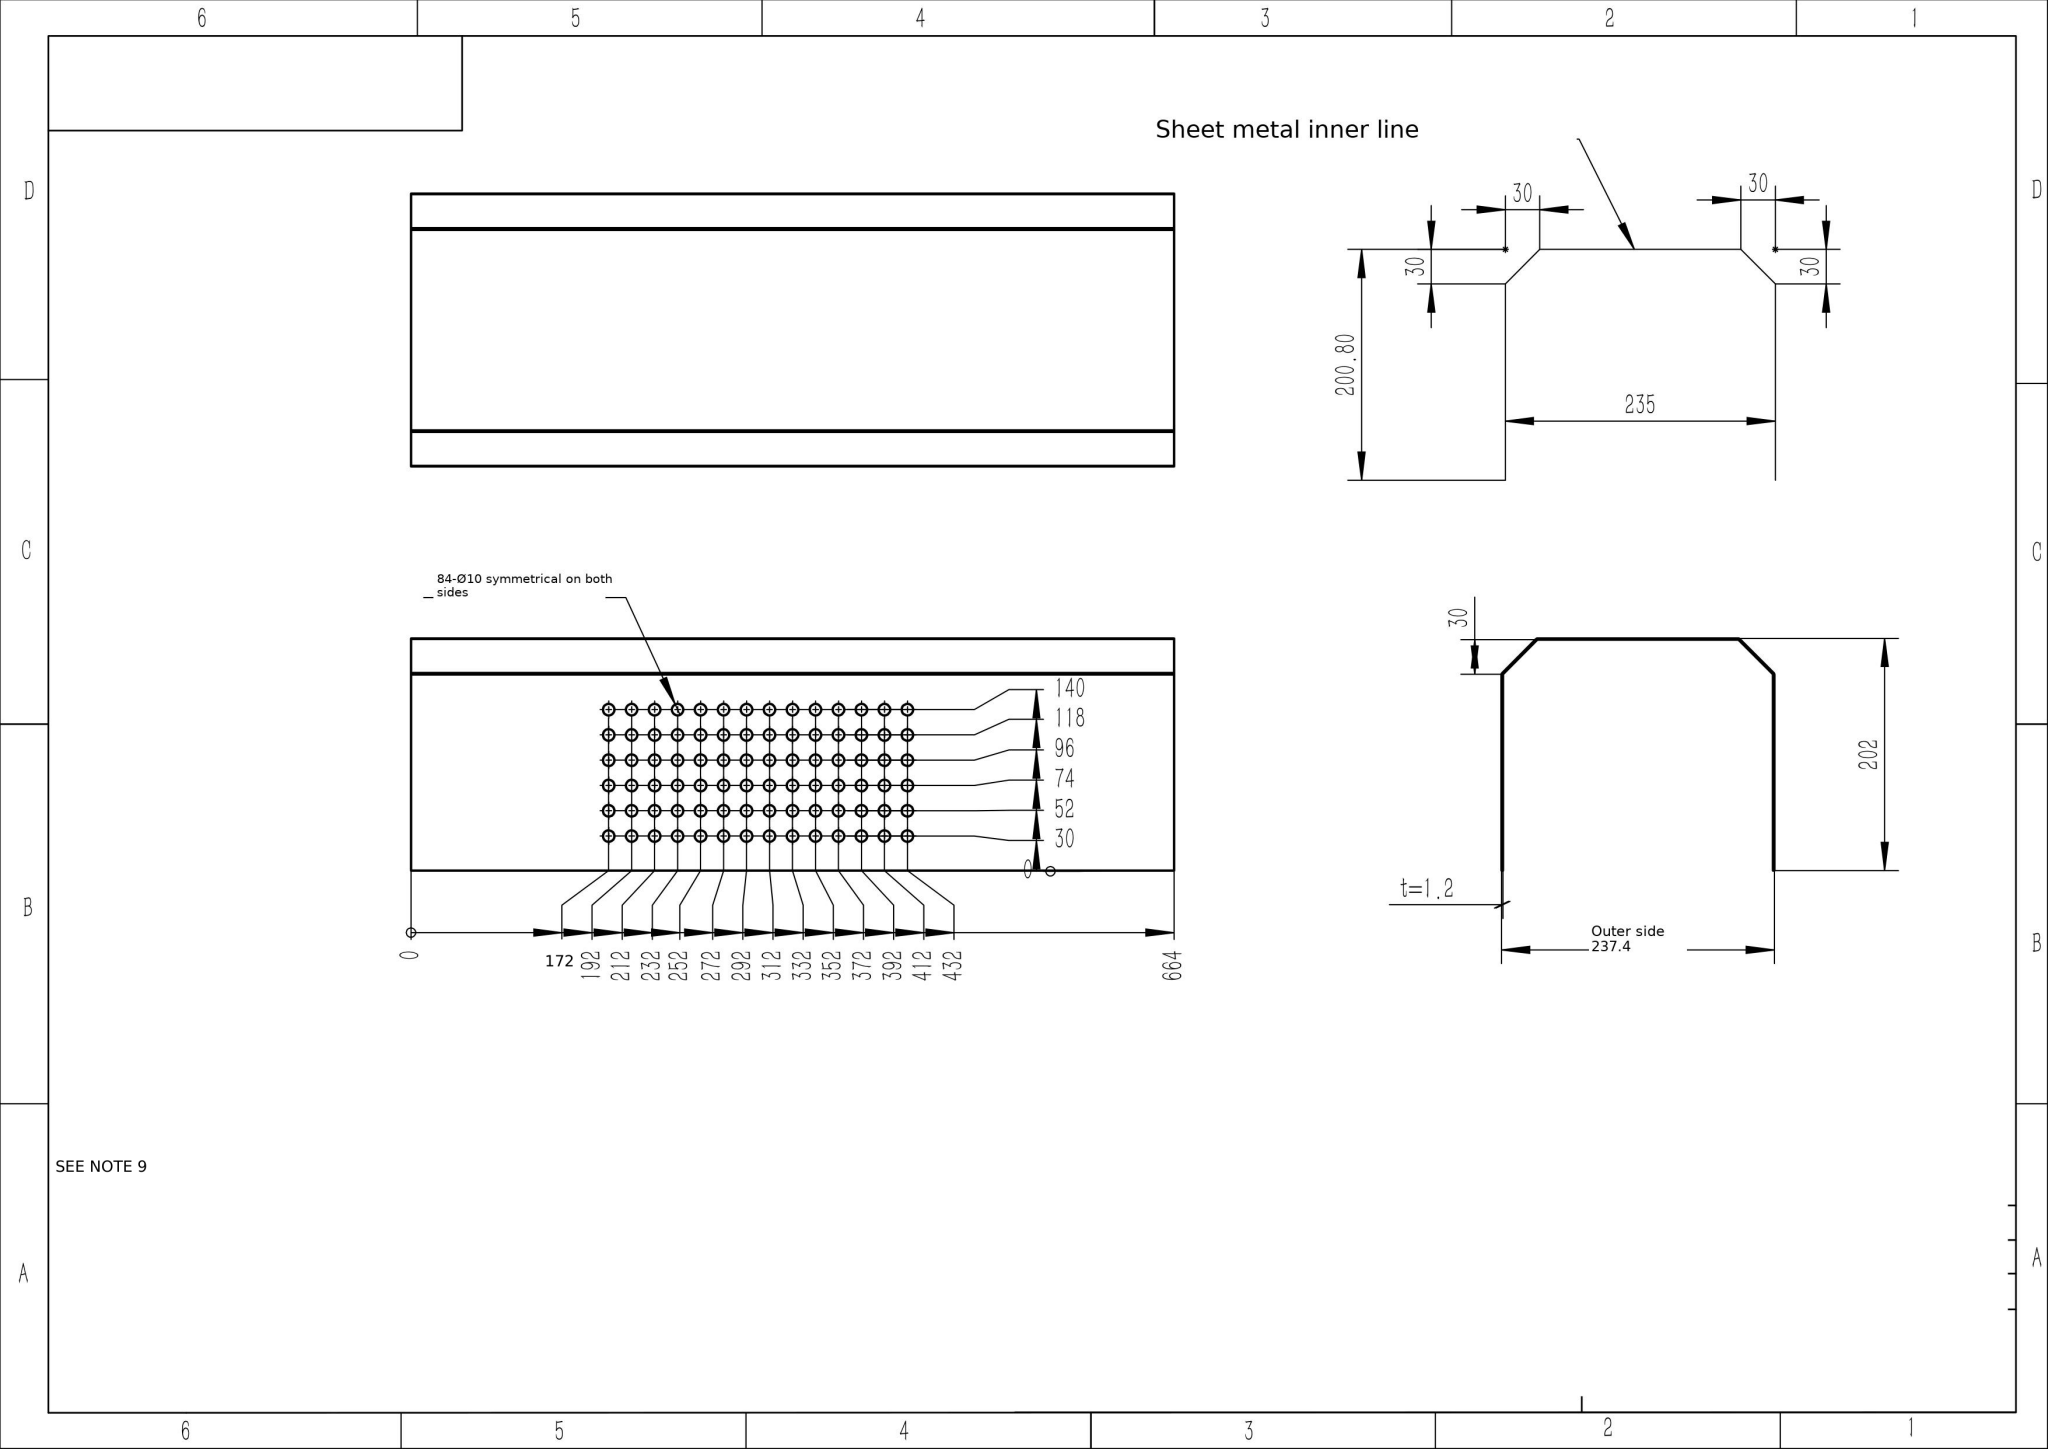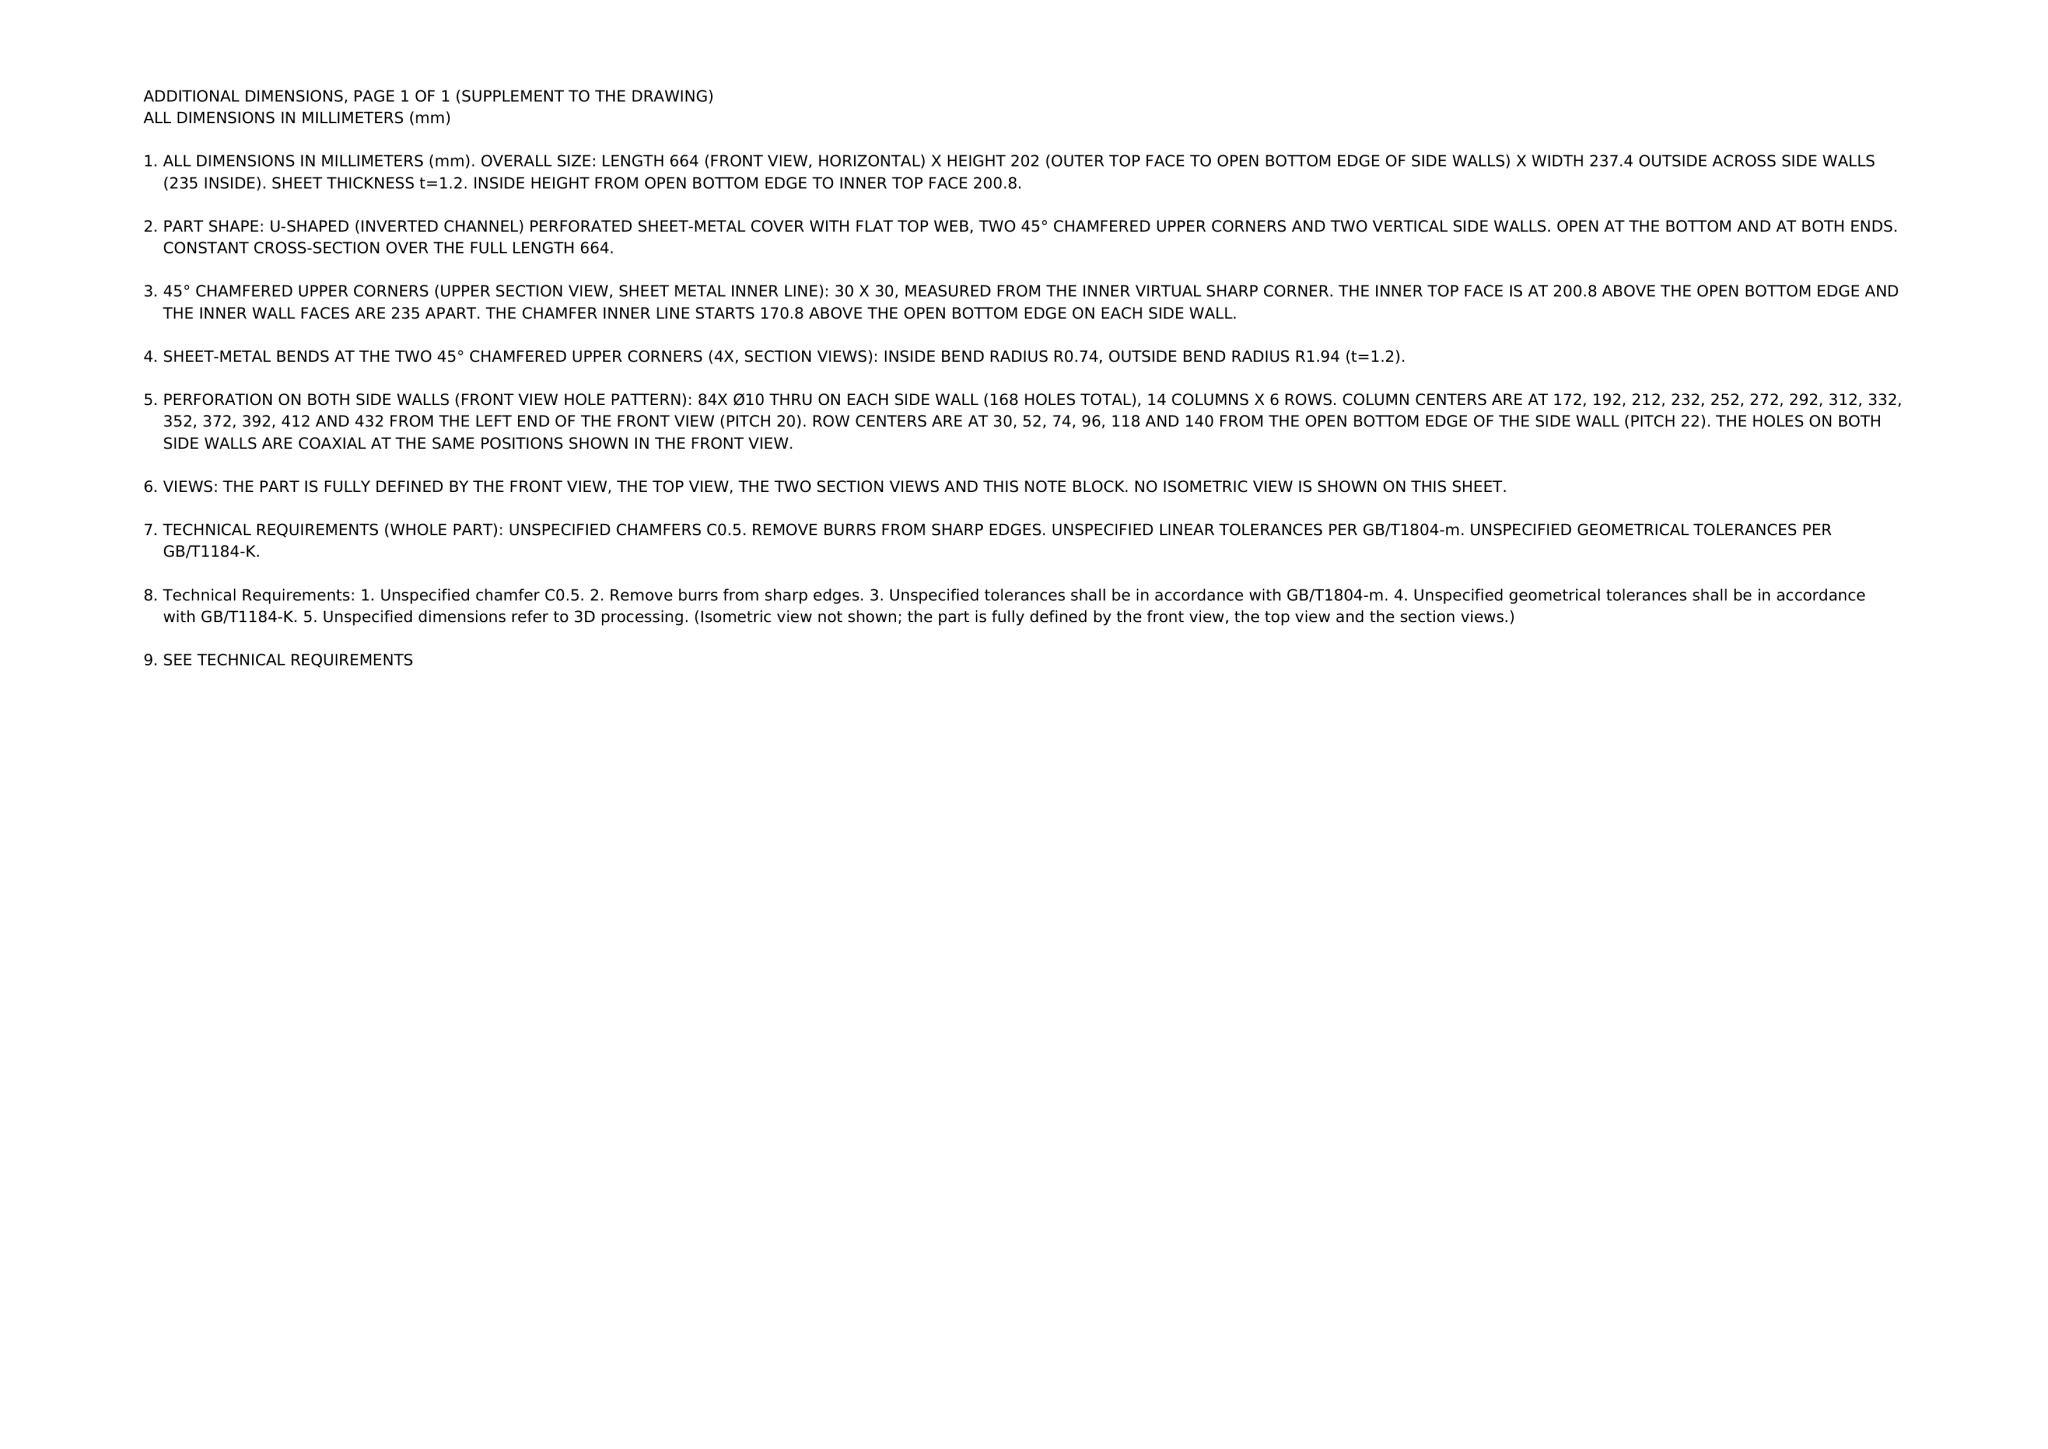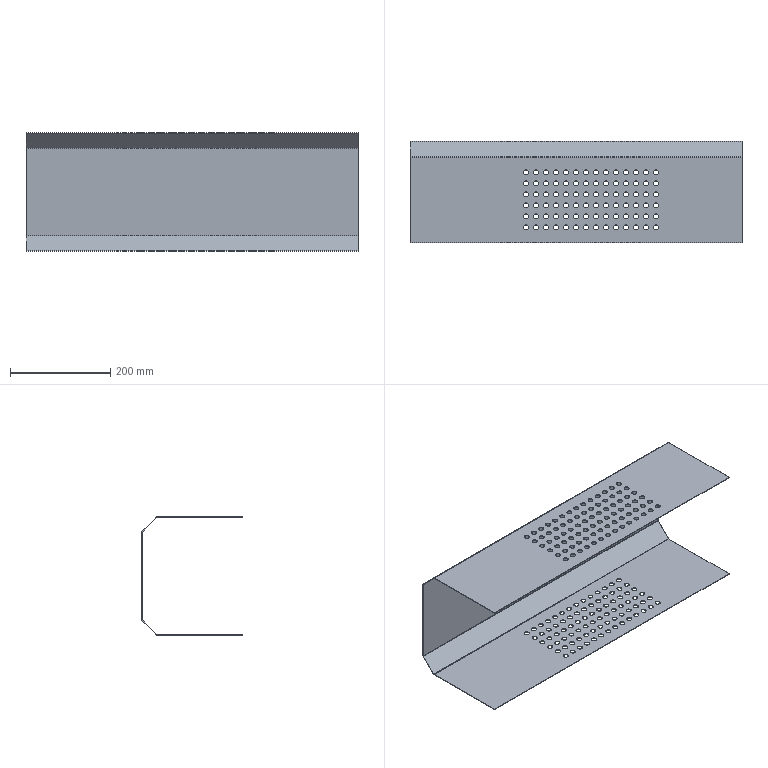Part | NX | mm | 1 solid | 374 faces | box 664 x 202 x 237.4 mm | volume 464805 mm3 | cylinder 344 | plane 30 | commonest cylinder face diameters 10 x336 1.473 x4 3.873 x4